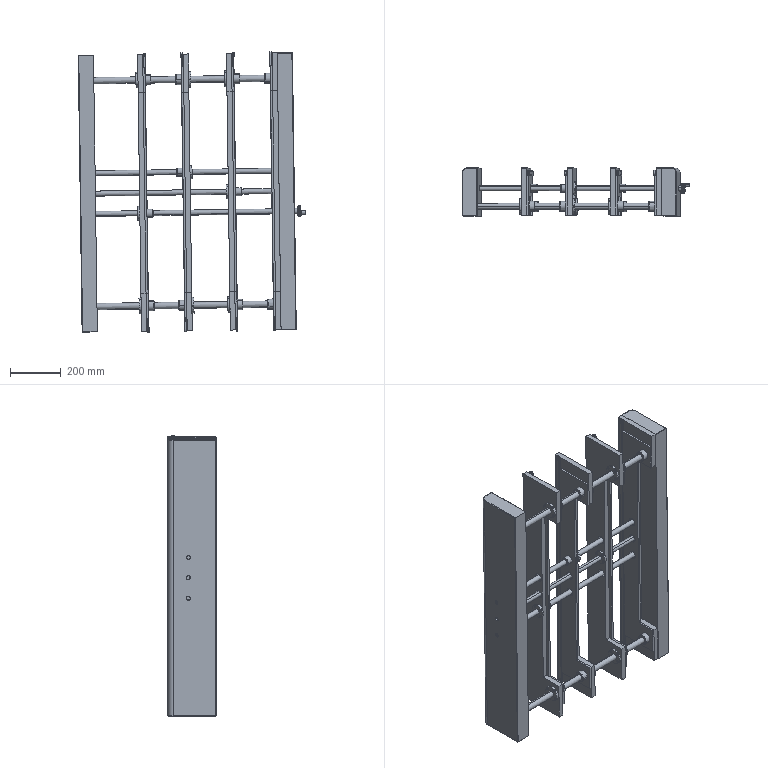Assembly | SolidWorks | mm | 39 component files | 39 solids | 1245 faces | box 896.58 x 189.84 x 1105.9 mm | volume 40372538 mm3 | plane 560 | cylinder 552 | cone 82 | spline 27 | torus 22 | sphere 2 | commonest cylinder face diameters 5.5 x88 9 x88 32 x54 40 x51 19 x36 18 x32 25 x24 4 x22
Bill of materials:
DA-0220-HBK40 | 1 |  | Knurled round knob: a wide disc with a straight-knurled rim, a plain cylindrical boss on one face, and a smaller cylindrical pin sticking out of the opposite face off-centre, near the rim.
DA-0220-LHFR20-1 | 3 |  | Flanged cylindrical sleeve: a long tubular body with a through bore and a round flange at one end with four through holes.
DA-0220-LHFR25 | 8 |  | Flanged cylindrical sleeve: like the previous part but with a shorter body. It has a round flange with four through holes and a central through bore.
DA-0220-Part10 | 4 |  | Thin flat bracket or strip: a long narrow plate with tabs at both ends extending to one side, giving a C-shaped outline. Each tab has one hole, and three small holes run in a line along the middle of the strip. A thin lip or flange appears along one long edge.
DA-0220-Part11 | 8 |  | Spool- or pulley-like rotational part: a cylindrical hub between two thin end flanges, with a plain central through bore.
DA-0220-Part15 | 2 |  | Plain solid cylindrical rod: long and slender with a constant diameter and flat ends.
DA-0220-Part16 | 4 |  | Very thin body that looks like a sheet in three views. One orthographic view shows a rectangular outline with a large central rectangular opening and banded shading on the side regions.
DA-0220-Part3 | 4 |  | Flat plate bracket: a long strip with tabs at both ends extending to one side, giving a C-shaped outline. Each tab has one hole, and three small holes run in a line along the strip. Similar outline to unnamed part but with no visible edge lip.
DA-0220-Part8 | 1 |  | Rectangular bar or block, longer than it is wide, with three small holes in a line along the centre of one face. One orthographic view shows a large rounded corner.
DA-0220-Part9 | 1 |  | Rectangular bar or block with three small holes in a line along the centre of one face. One view shows a rounded corner on the opposite side compared with unnamed part.
DA-0220-Screw | 3 |  | Long slender stepped shaft: a main cylindrical body with a short smaller-diameter journal at each end.
Mates:
1. distance | DA-0220-Part3-1 face at (503.745, -113.85, -534.522) dir (0.9999, 0.000404, 0.01395) | DA-0220-Part3-2 face at (663.729, -113.786, -532.29) dir (-0.9999, -0.000404, -0.01395)
2. coincident | DA-0220-Part3-1 face at (488.494, -13.853, 555.371) dir (-0.000404, 1, -0.00000282) | DA-0220-Part3-2 face at (668.477, -13.781, 557.883) dir (-0.000404, 1, -0.00000282)
3. coincident | DA-0220-Part3-1 face at (503.704, -13.85, -534.523) dir (0.01395, 0.00000282, -0.9999) | DA-0220-Part3-2 face at (683.687, -13.778, -532.011) dir (0.01395, 0.00000282, -0.9999)
4. coincident | DA-0220-Part3-2 face at (668.477, -13.781, 557.883) dir (-0.01395, -0.00000282, 0.9999) | DA-0220-Part3-3 face at (838.46, -13.712, 560.255) dir (-0.01395, -0.00000282, 0.9999)
5. coincident | DA-0220-Part3-2 face at (668.477, -13.781, 557.883) dir (-0.000404, 1, -0.00000282) | DA-0220-Part3-3 face at (838.46, -13.712, 560.255) dir (-0.000404, 1, -0.00000282)
6. distance | DA-0220-Part3-4 face at (1013.695, -113.644, -527.406) dir (-0.9999, -0.000404, -0.01395) | DA-0220-Part3-3 face at (853.711, -113.709, -529.639) dir (0.9999, 0.000404, 0.01395)
7. coincident | DA-0220-Part3-1 face at (483.747, -113.858, -534.802) dir (-0.9999, -0.000404, -0.01395) | DA-0220-LHFR25-3 face at (470.145, -186.546, 441.974) dir (0.9999, 0.000404, 0.01395)
8. coincident | DA-0220-Part3-3 face at (833.713, -113.717, -529.918) dir (-0.9999, -0.000404, -0.01395) | DA-0220-LHFR25-18 face at (820.141, -184.786, 444.602) dir (0.9999, 0.000404, 0.01395)
9. coincident | DA-0220-Part3-4 face at (1033.693, -113.636, -527.127) dir (0.9999, 0.000404, 0.01395) | DA-0220-LHFR25-20 face at (1019.619, -179.113, 483.237) dir (-0.9999, -0.000404, -0.01395)
10. coincident | DA-0220-Part3-4 face at (1013.695, -113.644, -527.406) dir (-0.9999, -0.000404, -0.01395) | DA-0220-Part10-3 face at (998.456, -41.647, 562.488) dir (0.9999, 0.000404, 0.01395)
11. coincident | DA-0220-Part11-7 face at (995.508, -35.862, 558.608) dir (0.9999, 0.000404, 0.01395) | DA-0220-Part11-13 face at (1010.577, -35.838, -521.247) dir (0.9999, 0.000404, 0.01395)
12. coincident | DA-0220-Part10-3 face at (1010.661, -27.646, -527.448) dir (-0.9999, -0.000404, -0.01395) | DA-0220-Part11-13 face at (1010.577, -35.838, -521.247) dir (0.9999, 0.000404, 0.01395)
13. concentric | DA-0220-Part11-7 face at (992.023, -33.65, 557.398) dir (-0.9999, -0.000404, -0.01395) r 7 | DA-0220-Part16-3 face at (989.523, -33.651, 557.363) dir (0.9999, 0.000404, 0.01395) r 9.5
14. concentric | DA-0220-Part11-13 face at (1007.094, -33.647, -522.497) dir (-0.9999, -0.000404, -0.01395) r 7 | DA-0220-Part16-3 face at (1004.594, -33.648, -522.532) dir (0.9999, 0.000404, 0.01395) r 8.25
15. coincident | DA-0220-Part11-13 face at (1009.536, -41.539, -518.138) dir (-0.9999, -0.000404, -0.01395) | DA-0220-Part16-3 face at (1009.593, -33.646, -522.462) dir (0.9999, 0.000404, 0.01395)
16. coincident | DA-0220-Part3-4 face at (1018.443, -13.639, 562.767) dir (-0.01395, -0.00000282, 0.9999) | DA-0220-Part9-4 face at (1018.519, -203.139, 562.767) dir (-0.01395, -0.00000282, 0.9999)
17. coincident | DA-0220-Part9-4 face at (1078.437, -13.615, 563.604) dir (0.9999, 0.000404, 0.01395) | DA-0220-HBK40-4 face at (1087.162, -98.389, -59.155) dir (-0.9999, -0.000404, -0.01395)
18. coincident | DA-0220-Part3-4 face at (1033.693, -113.636, -527.127) dir (0.9999, 0.000404, 0.01395) | DA-0220-Part9-4 face at (1018.519, -203.139, 562.767) dir (-0.9999, -0.000404, -0.01395)
19. distance | DA-0220-Part3-1 face at (503.745, -113.85, -534.522) dir (0.9999, 0.000404, 0.01395) | DA-0220-Part3-3 face at (853.711, -113.709, -529.639) dir (0.9999, 0.000404, 0.01395)
20. coincident | DA-0220-Screw-4 face at (1026.168, -89.779, 11.389) dir (0.9999, 0.000404, 0.01395) | DA-0220-Screw-8 face at (1027.262, -99.601, -66.719) dir (0.9999, 0.000404, 0.01395)
21. coincident | DA-0220-Screw-4 face at (1026.168, -89.779, 11.389) dir (0.9999, 0.000404, 0.01395) | DA-0220-Screw-7 face at (1024.875, -89.511, 104.074) dir (0.9999, 0.000404, 0.01395)
22. concentric | DA-0220-Part3-2 face at (655, -93.787, 92.649) dir (0.9999, 0.000404, 0.01395) r 16 | DA-0220-LHFR20-1-16 face at (682.997, -93.776, 93.04) dir (-0.9999, -0.000404, -0.01395) r 16
23. coincident | DA-0220-Part3-2 face at (683.727, -113.778, -532.011) dir (0.9999, 0.000404, 0.01395) | DA-0220-LHFR20-1-16 face at (674.808, -98.081, 106.67) dir (-0.9999, -0.000404, -0.01395)
24. coincident | DA-0220-Part3-1 face at (483.747, -113.858, -534.802) dir (-0.9999, -0.000404, -0.01395) | DA-0220-LHFR20-1-15 face at (477.374, -82.765, -79.025) dir (0.9999, 0.000404, 0.01395)
25. concentric | DA-0220-Screw-8 face at (249.272, -93.952, -73.028) dir (0.9999, 0.000404, 0.01395) r 10 | DA-0220-LHFR20-1-15 face at (469.251, -93.863, -69.958) dir (-0.9999, -0.000404, -0.01395) r 10
26. concentric | DA-0220-Part9-4 face at (1026.08, -93.638, 17.82) dir (0.9999, 0.000404, 0.01395) r 8 | DA-0220-Screw-4 face at (248.156, -93.952, 6.964) dir (0.9999, 0.000404, 0.01395) r 10
27. concentric | DA-0220-Part15-1 face at (295.97, -165.932, 452.674) dir (0.9999, 0.000404, 0.01395) r 12.5 | DA-0220-LHFR25-18 face at (844.817, -165.71, 460.334) dir (0.9999, 0.000404, 0.01395) r 20
28. concentric | DA-0220-Part9-4 face at (1024.964, -93.638, 97.812) dir (0.9999, 0.000404, 0.01395) r 8 | DA-0220-Screw-7 face at (247.04, -93.952, 86.956) dir (0.9999, 0.000404, 0.01395) r 10
29. coincident | DA-0220-Part3-4 face at (1018.443, -13.639, 562.767) dir (-0.000404, 1, -0.00000282) | DA-0220-Part9-4 face at (1018.443, -13.639, 562.767) dir (-0.000404, 1, -0.00000282)
30. coincident | DA-0220-Part3-3 face at (853.67, -13.709, -529.639) dir (0.01395, 0.00000282, -0.9999) | DA-0220-Part3-4 face at (1033.653, -13.636, -527.127) dir (0.01395, 0.00000282, -0.9999)
31. coincident | DA-0220-Part3-3 face at (838.46, -13.712, 560.255) dir (-0.000404, 1, -0.00000282) | DA-0220-Part3-4 face at (1018.443, -13.639, 562.767) dir (-0.000404, 1, -0.00000282)
32. coincident | DA-0220-Part9-4 face at (1018.443, -13.639, 562.767) dir (-0.000404, 1, -0.00000282) | DA-0220-Part8-5 face at (309.723, -13.929, -537.23) dir (-0.000404, 1, -0.00000282)
33. concentric | DA-0220-Part10-3 face at (995.523, -33.649, 557.446) dir (-0.9999, -0.000404, -0.01395) r 2.1 | DA-0220-Part11-7 face at (992.023, -33.65, 557.398) dir (-0.9999, -0.000404, -0.01395) r 2.5
34. concentric | DA-0220-Part10-3 face at (1010.593, -33.646, -522.448) dir (-0.9999, -0.000404, -0.01395) r 2.1 | DA-0220-Part11-13 face at (1007.094, -33.647, -522.497) dir (-0.9999, -0.000404, -0.01395) r 2.5
35. width | DA-0220-Part3-4 face at (1018.443, -13.639, 562.767) dir (-0.01395, -0.00000282, 0.9999) | DA-0220-Part3-4 face at (1033.653, -13.636, -527.127) dir (0.01395, 0.00000282, -0.9999) | DA-0220-Part10-3 face at (991.154, -41.65, 512.381) dir (-0.01395, -0.00000282, 0.9999) | DA-0220-Part10-3 face at (1005.003, -125.648, -477.522) dir (0.01395, 0.00000282, -0.9999)
36. concentric | DA-0220-Part3-4 face at (1007.198, -93.646, -62.451) dir (0.9999, 0.000404, 0.01395) r 16 | DA-0220-Screw-8 face at (249.272, -93.952, -73.028) dir (0.9999, 0.000404, 0.01395) r 10
37. coincident | DA-0220-Screw-7 face at (300.915, -88.428, 96.059) dir (-0.9999, -0.000404, -0.01395) | DA-0220-Part8-5 face at (309.8, -203.429, -537.229) dir (0.9999, 0.000404, 0.01395)
38. concentric | DA-0220-Part3-1 face at (469.953, -165.861, 455.102) dir (0.9999, 0.000404, 0.01395) r 20 | DA-0220-LHFR25-3 face at (494.851, -165.851, 455.45) dir (0.9999, 0.000404, 0.01395) r 20
39. concentric | DA-0220-Part3-2 face at (649.936, -165.788, 457.614) dir (0.9999, 0.000404, 0.01395) r 20 | DA-0220-LHFR25-22 face at (645.036, -165.79, 457.546) dir (-0.9999, -0.000404, -0.01395) r 20
40. coincident | DA-0220-Part3-2 face at (683.727, -113.778, -532.011) dir (0.9999, 0.000404, 0.01395) | DA-0220-LHFR25-22 face at (670.274, -163.832, 433.473) dir (-0.9999, -0.000404, -0.01395)
41. concentric | DA-0220-Part3-3 face at (819.919, -165.72, 459.986) dir (0.9999, 0.000404, 0.01395) r 20 | DA-0220-LHFR25-18 face at (844.817, -165.71, 460.334) dir (0.9999, 0.000404, 0.01395) r 20
42. concentric | DA-0220-Part3-4 face at (999.901, -165.647, 462.498) dir (0.9999, 0.000404, 0.01395) r 20 | DA-0220-LHFR25-20 face at (995.002, -165.649, 462.429) dir (-0.9999, -0.000404, -0.01395) r 20
43. coincident | DA-0220-Part15-1 face at (295.97, -165.932, 452.674) dir (-0.9999, -0.000404, -0.01395) | DA-0220-Part8-5 face at (309.8, -203.429, -537.229) dir (0.9999, 0.000404, 0.01395)
44. distance | DA-0220-Part10-3 face at (1005.66, -25.648, -527.518) dir (-0.000404, 1, -0.00000282) | DA-0220-Part3-4 face at (1018.443, -13.639, 562.767) dir (-0.000404, 1, -0.00000282)
45. concentric | DA-0220-Screw-4 face at (248.156, -93.952, 6.964) dir (0.9999, 0.000404, 0.01395) r 10 | DA-0220-Part8-5 face at (302.151, -93.93, 7.717) dir (-0.9999, -0.000404, -0.01395) r 8
46. coincident | DA-0220-Part9-4 face at (1018.519, -203.139, 562.767) dir (-0.9999, -0.000404, -0.01395) | DA-0220-Screw-7 face at (1024.875, -89.511, 104.074) dir (0.9999, 0.000404, 0.01395)
47. concentric | DA-0220-HBK40-4 face at (1093.69, -93.611, -61.244) dir (-0.9999, -0.000404, -0.01395) r 11 | DA-0220-Screw-8 face at (249.272, -93.952, -73.028) dir (0.9999, 0.000404, 0.01395) r 10
48. concentric | DA-0220-LHFR20-1-6 face at (818.1, -93.722, 14.918) dir (0.9999, 0.000404, 0.01395) r 16 | DA-0220-Screw-4 face at (248.156, -93.952, 6.964) dir (0.9999, 0.000404, 0.01395) r 10